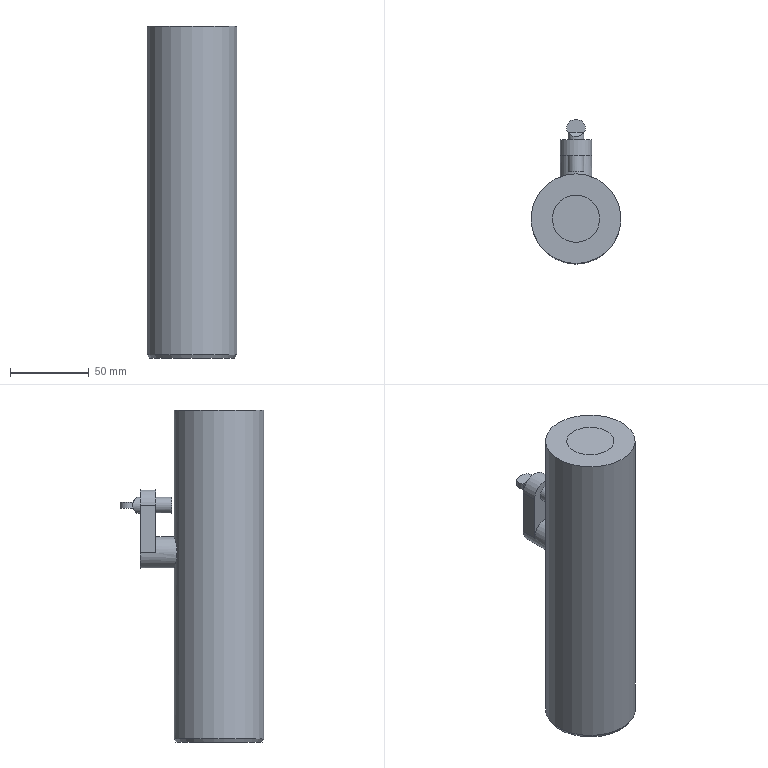Component | NX | 12 | 2 solids | 26 faces | volume 484638 mm3 | plane 15 | cylinder 10 | cone 1 | commonest cylinder face diameters 10 x4 20 x3 30 x2 56.9 x1